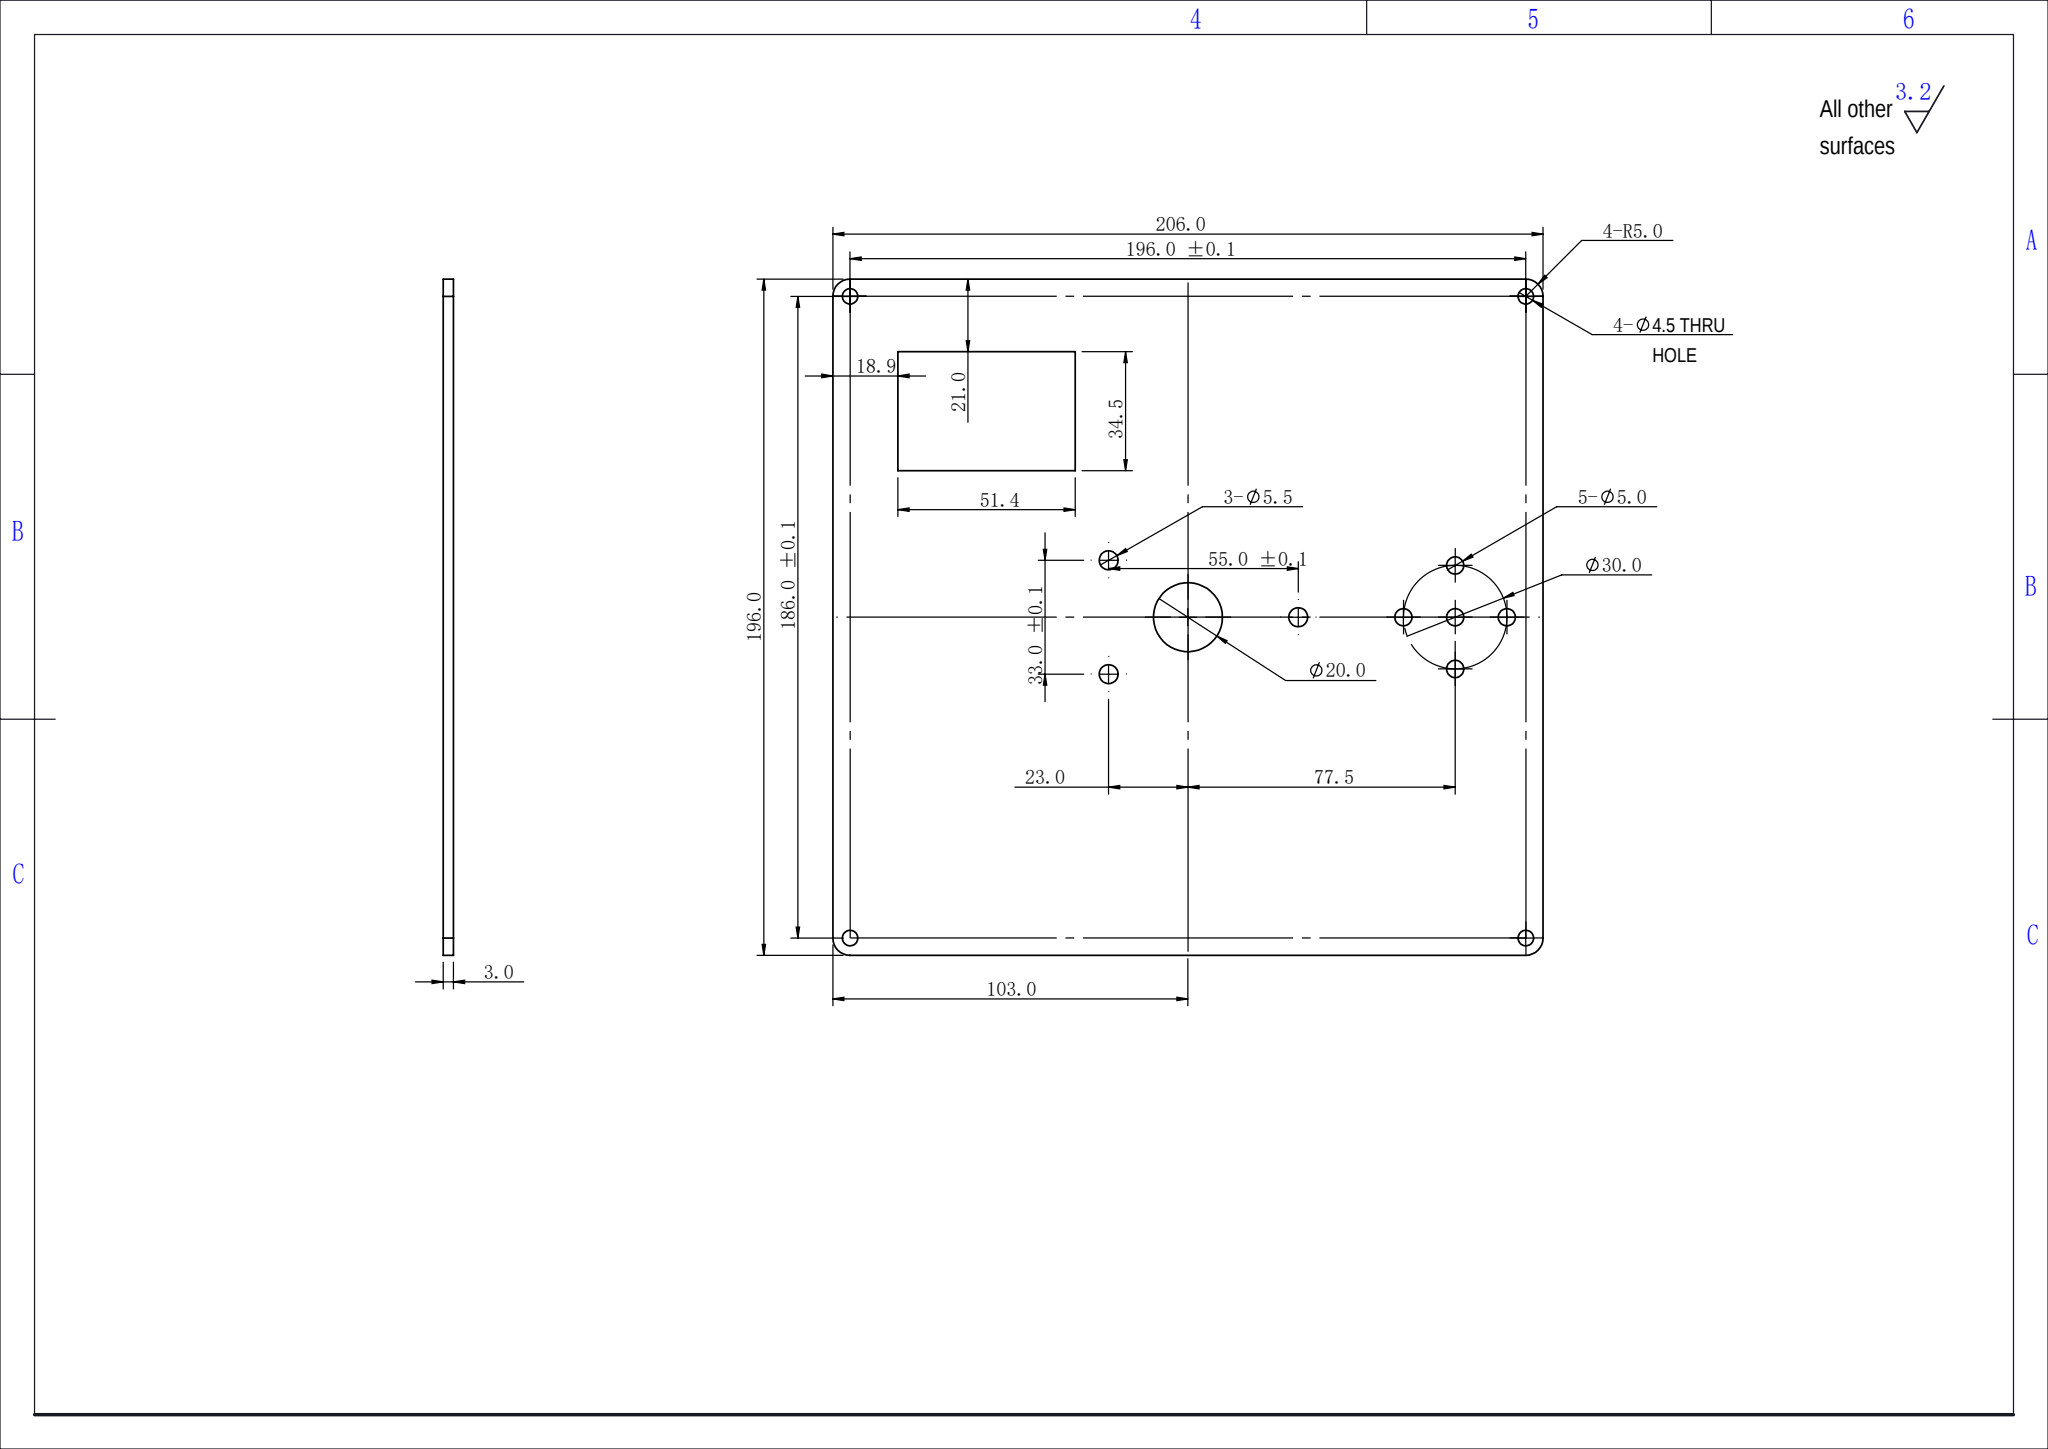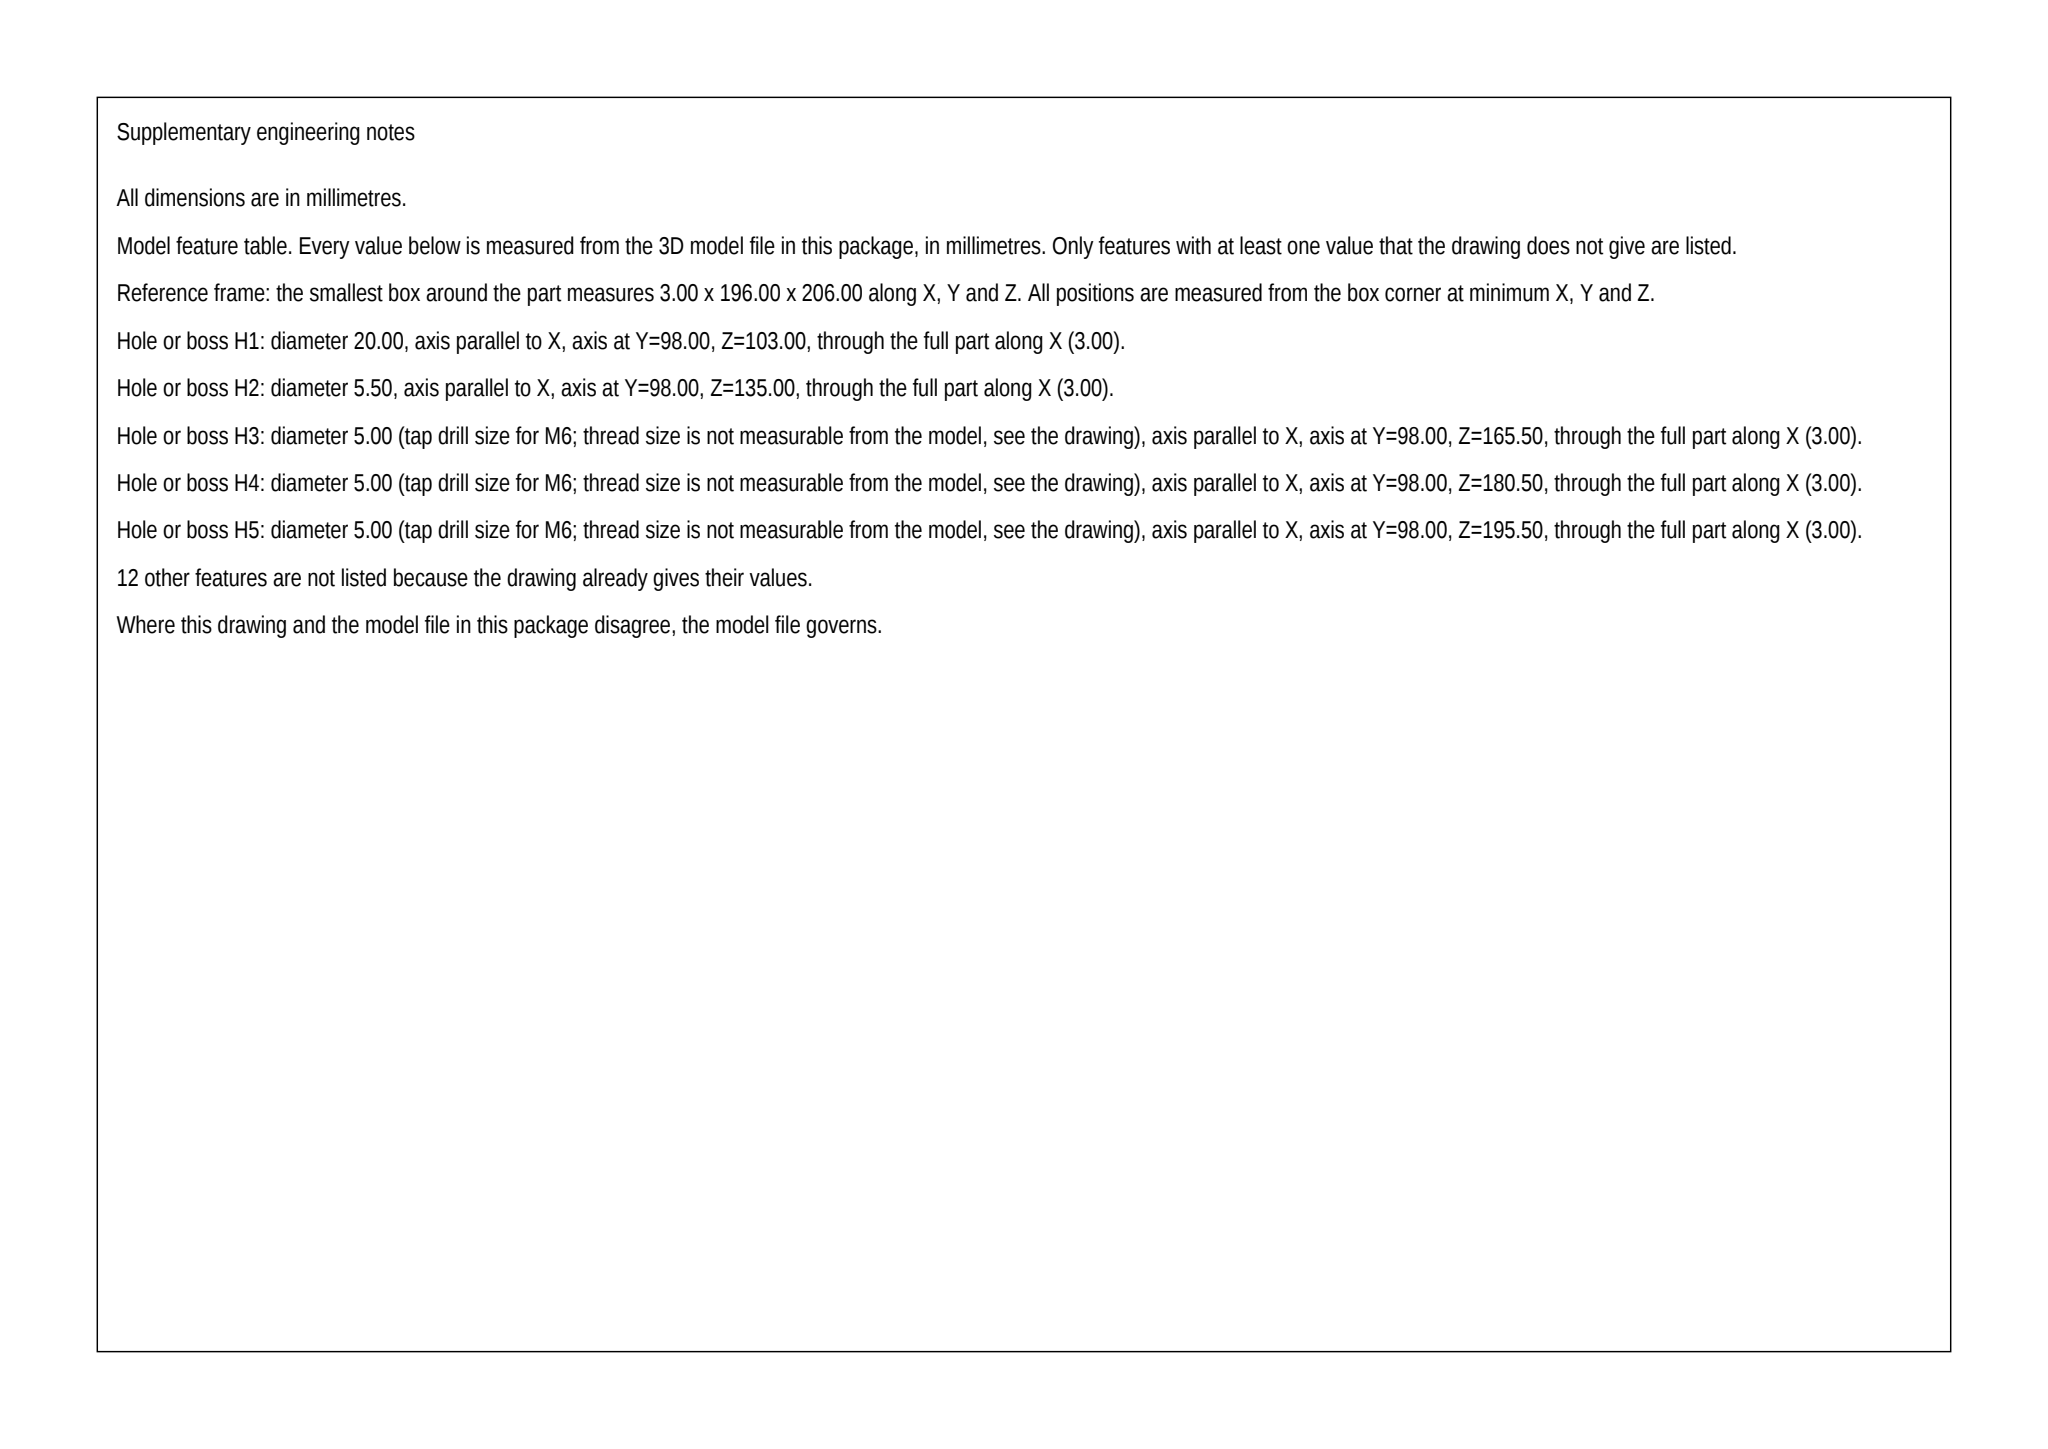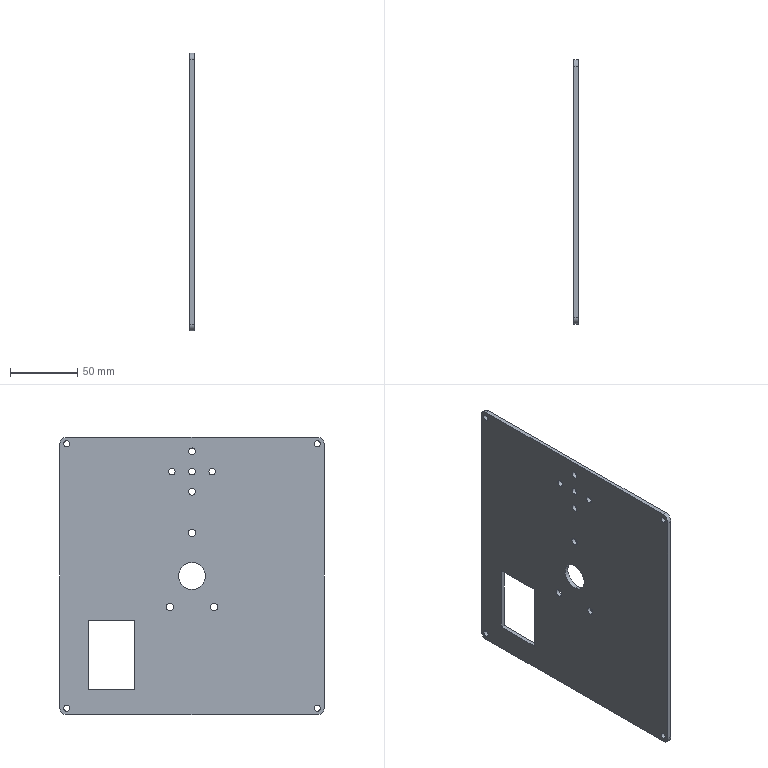Part | SolidWorks | mm | 1 solid | 40 faces | box 3 x 196 x 206 mm | volume 114101 mm3 | cylinder 30 | plane 10 | commonest cylinder face diameters 5 x10 4.5 x8 5.5 x6 10 x4 20 x2